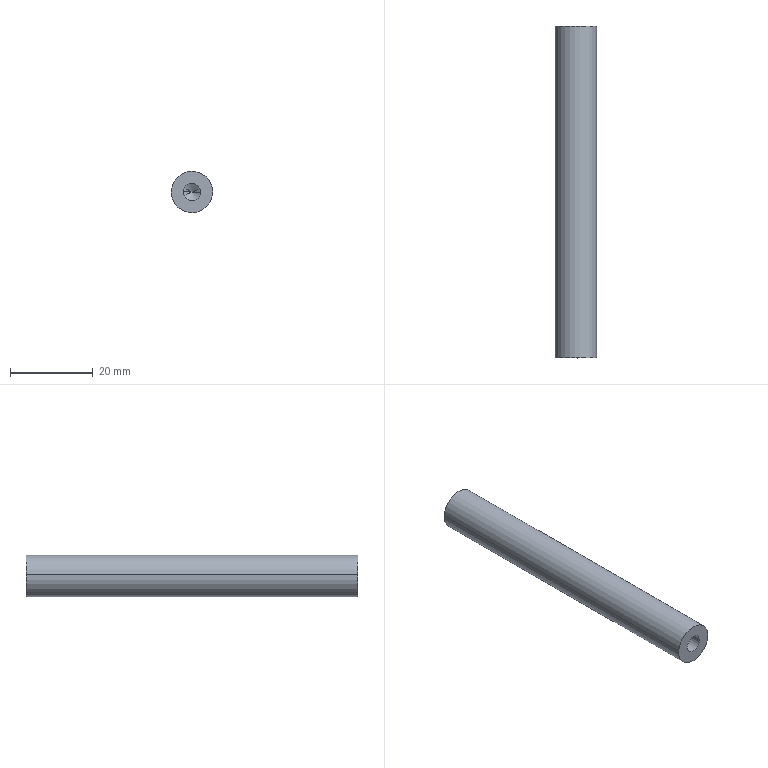Component | SolidWorks | 75-02-22MotorConnectingRod-1 | 1 solid | 12 faces | box 10 x 80 x 10 mm | volume 5928 mm3 | cylinder 6 | cone 4 | plane 2 | commonest cylinder face diameters 4.2 x4 10 x2 | material A3 Steel
build123d program:
from build123d import *

# Parameters (mm, degrees)
SKETCH1_R                       = 5
BOSS_EXTRUDE1_DEPTH             = 40
M5_TAPPED_HOLE1_D               = 4.2
M5_TAPPED_HOLE1_DEPTH           = 12.4
M5_TAPPED_HOLE1_TIP             = 1.262
M5_TAPPED_HOLE1_ON_FACE_2_D     = 4.2
M5_TAPPED_HOLE1_ON_FACE_2_DEPTH = 12.4
M5_TAPPED_HOLE1_ON_FACE_2_TIP   = 1.262


with BuildPart() as part:
    # Sketch1 → Boss-Extrude1 (new, symmetric)
    with BuildSketch(Plane.XY):
        Circle(SKETCH1_R)
    extrude(amount=BOSS_EXTRUDE1_DEPTH, both=True)

    # M5 Tapped Hole1
    with Locations(Plane.XY.offset(40)):
        with Locations((0, 0)):
            Hole(M5_TAPPED_HOLE1_D / 2, depth=M5_TAPPED_HOLE1_DEPTH)
            with Locations((0, 0, -(M5_TAPPED_HOLE1_DEPTH + M5_TAPPED_HOLE1_TIP / 2))):  # 118° drill point
                Cone(0, M5_TAPPED_HOLE1_D / 2, M5_TAPPED_HOLE1_TIP, mode=Mode.SUBTRACT)

    # M5 Tapped Hole1 on face 2
    with Locations(Plane(origin=(0, 0, -40), x_dir=(-1, 0, 0), z_dir=(0, 0, -1))):
        with Locations((0, 0)):
            Hole(M5_TAPPED_HOLE1_ON_FACE_2_D / 2, depth=M5_TAPPED_HOLE1_ON_FACE_2_DEPTH)
            with Locations((0, 0, -(M5_TAPPED_HOLE1_ON_FACE_2_DEPTH + M5_TAPPED_HOLE1_ON_FACE_2_TIP / 2))):  # 118° drill point
                Cone(0, M5_TAPPED_HOLE1_ON_FACE_2_D / 2, M5_TAPPED_HOLE1_ON_FACE_2_TIP, mode=Mode.SUBTRACT)


solid = part.part

# Placed as in the assembly
solid = solid.moved(Location((-17.8, 155.857, -17.75), (90, 0, 0)))
STEP:
#1=CARTESIAN_POINT('',(-0.6183,5.049,-0.7045));
#2=VERTEX_POINT('',#1);
#3=CARTESIAN_POINT('',(-0.7833,5.049,-0.6931));
#4=VERTEX_POINT('',#3);
#5=CARTESIAN_POINT('',(-0.7008,5.049,-0.6988));
#6=DIRECTION('',(-0.,-1.,0.));
#7=DIRECTION('',(-0.9976,0.,0.06881));
#8=AXIS2_PLACEMENT_3D('',#5,#6,#7);
#9=CIRCLE('',#8,0.08268);
#10=EDGE_CURVE('',#2,#4,#9,.T.);
#11=ORIENTED_EDGE('',*,*,#10,.F.);
#12=CARTESIAN_POINT('',(-0.6183,4.561,-0.7045));
#13=VERTEX_POINT('',#12);
#14=CARTESIAN_POINT('',(-0.6183,4.561,-0.7045));
#15=DIRECTION('',(-0.,-1.,0.));
#16=VECTOR('',#15,39.37);
#17=LINE('',#14,#16);
#18=EDGE_CURVE('',#2,#13,#17,.T.);
#19=ORIENTED_EDGE('',*,*,#18,.T.);
#20=CARTESIAN_POINT('',(-0.7833,4.561,-0.6931));
#21=VERTEX_POINT('',#20);
#22=CARTESIAN_POINT('',(-0.7008,4.561,-0.6988));
#23=DIRECTION('',(-0.,-1.,0.));
#24=DIRECTION('',(-0.9976,0.,0.06881));
#25=AXIS2_PLACEMENT_3D('',#22,#23,#24);
#26=CIRCLE('',#25,0.08268);
#27=EDGE_CURVE('',#13,#21,#26,.T.);
#28=ORIENTED_EDGE('',*,*,#27,.T.);
#29=CARTESIAN_POINT('',(-0.7833,4.561,-0.6931));
#30=DIRECTION('',(-0.,-1.,0.));
#31=VECTOR('',#30,39.37);
#32=LINE('',#29,#31);
#33=EDGE_CURVE('',#4,#21,#32,.T.);
#34=ORIENTED_EDGE('',*,*,#33,.F.);
#35=EDGE_LOOP('',(#11,#19,#28,#34));
#36=FACE_OUTER_BOUND('',#35,.T.);
#37=CARTESIAN_POINT('',(-0.7008,4.561,-0.6988));
#38=DIRECTION('',(-0.,-1.,0.));
#39=DIRECTION('',(-0.9976,0.,0.06881));
#40=AXIS2_PLACEMENT_3D('',#37,#38,#39);
#41=CYLINDRICAL_SURFACE('',#40,0.08268);
#42=ADVANCED_FACE('',(#36),#41,.F.);
#43=CARTESIAN_POINT('',(-0.7008,5.099,-0.6988));
#44=VERTEX_POINT('',#43);
#45=CARTESIAN_POINT('',(-0.7833,5.049,-0.6931));
#46=DIRECTION('',(-0.8551,-0.515,0.05899));
#47=VECTOR('',#46,39.37);
#48=LINE('',#45,#47);
#49=EDGE_CURVE('',#44,#4,#48,.T.);
#50=ORIENTED_EDGE('',*,*,#49,.F.);
#51=CARTESIAN_POINT('',(-0.6183,5.049,-0.7045));
#52=DIRECTION('',(0.8551,-0.515,-0.05899));
#53=VECTOR('',#52,39.37);
#54=LINE('',#51,#53);
#55=EDGE_CURVE('',#44,#2,#54,.T.);
#56=ORIENTED_EDGE('',*,*,#55,.T.);
#57=ORIENTED_EDGE('',*,*,#10,.T.);
#58=EDGE_LOOP('',(#50,#56,#57));
#59=FACE_OUTER_BOUND('',#58,.T.);
#60=CARTESIAN_POINT('',(-0.7008,5.049,-0.6988));
#61=DIRECTION('',(-0.,-1.,0.));
#62=DIRECTION('',(-0.9976,0.,0.06881));
#63=AXIS2_PLACEMENT_3D('',#60,#61,#62);
#64=CONICAL_SURFACE('',#63,0.08268,1.03);
#65=ADVANCED_FACE('',(#59),#64,.F.);
#66=CARTESIAN_POINT('',(-0.7833,7.223,-0.6931));
#67=VERTEX_POINT('',#66);
#68=CARTESIAN_POINT('',(-0.6183,7.223,-0.7045));
#69=VERTEX_POINT('',#68);
#70=CARTESIAN_POINT('',(-0.7008,7.223,-0.6988));
#71=DIRECTION('',(0.,1.,-0.));
#72=DIRECTION('',(0.9976,0.,-0.06881));
#73=AXIS2_PLACEMENT_3D('',#70,#71,#72);
#74=CIRCLE('',#73,0.08268);
#75=EDGE_CURVE('',#67,#69,#74,.T.);
#76=ORIENTED_EDGE('',*,*,#75,.F.);
#77=CARTESIAN_POINT('',(-0.7833,7.711,-0.6931));
#78=VERTEX_POINT('',#77);
#79=CARTESIAN_POINT('',(-0.7833,7.711,-0.6931));
#80=DIRECTION('',(0.,1.,-0.));
#81=VECTOR('',#80,39.37);
#82=LINE('',#79,#81);
#83=EDGE_CURVE('',#67,#78,#82,.T.);
#84=ORIENTED_EDGE('',*,*,#83,.T.);
#85=CARTESIAN_POINT('',(-0.6183,7.711,-0.7045));
#86=VERTEX_POINT('',#85);
#87=CARTESIAN_POINT('',(-0.7008,7.711,-0.6988));
#88=DIRECTION('',(0.,1.,-0.));
#89=DIRECTION('',(0.9976,0.,-0.06881));
#90=AXIS2_PLACEMENT_3D('',#87,#88,#89);
#91=CIRCLE('',#90,0.08268);
#92=EDGE_CURVE('',#78,#86,#91,.T.);
#93=ORIENTED_EDGE('',*,*,#92,.T.);
#94=CARTESIAN_POINT('',(-0.6183,7.711,-0.7045));
#95=DIRECTION('',(0.,1.,-0.));
#96=VECTOR('',#95,39.37);
#97=LINE('',#94,#96);
#98=EDGE_CURVE('',#69,#86,#97,.T.);
#99=ORIENTED_EDGE('',*,*,#98,.F.);
#100=EDGE_LOOP('',(#76,#84,#93,#99));
#101=FACE_OUTER_BOUND('',#100,.T.);
#102=CARTESIAN_POINT('',(-0.7008,7.711,-0.6988));
#103=DIRECTION('',(0.,1.,-0.));
#104=DIRECTION('',(0.9976,0.,-0.06881));
#105=AXIS2_PLACEMENT_3D('',#102,#103,#104);
#106=CYLINDRICAL_SURFACE('',#105,0.08268);
#107=ADVANCED_FACE('',(#101),#106,.F.);
#108=CARTESIAN_POINT('',(-0.7008,7.173,-0.6988));
#109=VERTEX_POINT('',#108);
#110=CARTESIAN_POINT('',(-0.6183,7.223,-0.7045));
#111=DIRECTION('',(0.8551,0.515,-0.05899));
#112=VECTOR('',#111,39.37);
#113=LINE('',#110,#112);
#114=EDGE_CURVE('',#109,#69,#113,.T.);
#115=ORIENTED_EDGE('',*,*,#114,.F.);
#116=CARTESIAN_POINT('',(-0.7833,7.223,-0.6931));
#117=DIRECTION('',(-0.8551,0.515,0.05899));
#118=VECTOR('',#117,39.37);
#119=LINE('',#116,#118);
#120=EDGE_CURVE('',#109,#67,#119,.T.);
#121=ORIENTED_EDGE('',*,*,#120,.T.);
#122=ORIENTED_EDGE('',*,*,#75,.T.);
#123=EDGE_LOOP('',(#115,#121,#122));
#124=FACE_OUTER_BOUND('',#123,.T.);
#125=CARTESIAN_POINT('',(-0.7008,7.223,-0.6988));
#126=DIRECTION('',(0.,1.,-0.));
#127=DIRECTION('',(0.9976,0.,-0.06881));
#128=AXIS2_PLACEMENT_3D('',#125,#126,#127);
#129=CONICAL_SURFACE('',#128,0.08268,1.03);
#130=ADVANCED_FACE('',(#124),#129,.F.);
#131=CARTESIAN_POINT('',(-0.8972,4.561,-0.6853));
#132=VERTEX_POINT('',#131);
#133=CARTESIAN_POINT('',(-0.5044,4.561,-0.7124));
#134=VERTEX_POINT('',#133);
#135=CARTESIAN_POINT('',(-0.7008,4.561,-0.6988));
#136=DIRECTION('',(-0.,-1.,0.));
#137=DIRECTION('',(-0.9976,0.,0.06881));
#138=AXIS2_PLACEMENT_3D('',#135,#136,#137);
#139=CIRCLE('',#138,0.1969);
#140=EDGE_CURVE('',#132,#134,#139,.T.);
#141=ORIENTED_EDGE('',*,*,#140,.F.);
#142=CARTESIAN_POINT('',(-0.8972,7.711,-0.6853));
#143=VERTEX_POINT('',#142);
#144=CARTESIAN_POINT('',(-0.8972,4.561,-0.6853));
#145=DIRECTION('',(0.,1.,-0.));
#146=VECTOR('',#145,39.37);
#147=LINE('',#144,#146);
#148=EDGE_CURVE('',#132,#143,#147,.T.);
#149=ORIENTED_EDGE('',*,*,#148,.T.);
#150=CARTESIAN_POINT('',(-0.5044,7.711,-0.7124));
#151=VERTEX_POINT('',#150);
#152=CARTESIAN_POINT('',(-0.7008,7.711,-0.6988));
#153=DIRECTION('',(-0.,-1.,0.));
#154=DIRECTION('',(-0.9976,0.,0.06881));
#155=AXIS2_PLACEMENT_3D('',#152,#153,#154);
#156=CIRCLE('',#155,0.1969);
#157=EDGE_CURVE('',#143,#151,#156,.T.);
#158=ORIENTED_EDGE('',*,*,#157,.T.);
#159=CARTESIAN_POINT('',(-0.5044,4.561,-0.7124));
#160=DIRECTION('',(0.,1.,-0.));
#161=VECTOR('',#160,39.37);
#162=LINE('',#159,#161);
#163=EDGE_CURVE('',#134,#151,#162,.T.);
#164=ORIENTED_EDGE('',*,*,#163,.F.);
#165=EDGE_LOOP('',(#141,#149,#158,#164));
#166=FACE_OUTER_BOUND('',#165,.T.);
#167=CARTESIAN_POINT('',(-0.7008,4.561,-0.6988));
#168=DIRECTION('',(0.,1.,-0.));
#169=DIRECTION('',(0.9976,0.,-0.06881));
#170=AXIS2_PLACEMENT_3D('',#167,#168,#169);
#171=CYLINDRICAL_SURFACE('',#170,0.1969);
#172=ADVANCED_FACE('',(#166),#171,.T.);
#173=ORIENTED_EDGE('',*,*,#148,.F.);
#174=CARTESIAN_POINT('',(-0.7008,4.561,-0.6988));
#175=DIRECTION('',(-0.,-1.,0.));
#176=DIRECTION('',(-0.9976,0.,0.06881));
#177=AXIS2_PLACEMENT_3D('',#174,#175,#176);
#178=CIRCLE('',#177,0.1969);
#179=EDGE_CURVE('',#134,#132,#178,.T.);
#180=ORIENTED_EDGE('',*,*,#179,.F.);
#181=ORIENTED_EDGE('',*,*,#163,.T.);
#182=CARTESIAN_POINT('',(-0.7008,7.711,-0.6988));
#183=DIRECTION('',(-0.,-1.,0.));
#184=DIRECTION('',(-0.9976,0.,0.06881));
#185=AXIS2_PLACEMENT_3D('',#182,#183,#184);
#186=CIRCLE('',#185,0.1969);
#187=EDGE_CURVE('',#151,#143,#186,.T.);
#188=ORIENTED_EDGE('',*,*,#187,.T.);
#189=EDGE_LOOP('',(#173,#180,#181,#188));
#190=FACE_OUTER_BOUND('',#189,.T.);
#191=CARTESIAN_POINT('',(-0.7008,4.561,-0.6988));
#192=DIRECTION('',(0.,1.,-0.));
#193=DIRECTION('',(0.9976,0.,-0.06881));
#194=AXIS2_PLACEMENT_3D('',#191,#192,#193);
#195=CYLINDRICAL_SURFACE('',#194,0.1969);
#196=ADVANCED_FACE('',(#190),#195,.T.);
#197=CARTESIAN_POINT('',(-0.7008,4.561,-0.6988));
#198=DIRECTION('',(-0.,-1.,0.));
#199=DIRECTION('',(-0.9976,0.,0.06881));
#200=AXIS2_PLACEMENT_3D('',#197,#198,#199);
#201=CIRCLE('',#200,0.08268);
#202=EDGE_CURVE('',#21,#13,#201,.T.);
#203=ORIENTED_EDGE('',*,*,#202,.F.);
#204=ORIENTED_EDGE('',*,*,#27,.F.);
#205=EDGE_LOOP('',(#203,#204));
#206=FACE_BOUND('',#205,.T.);
#207=ORIENTED_EDGE('',*,*,#179,.T.);
#208=ORIENTED_EDGE('',*,*,#140,.T.);
#209=EDGE_LOOP('',(#207,#208));
#210=FACE_OUTER_BOUND('',#209,.T.);
#211=CARTESIAN_POINT('',(-0.7008,4.561,-0.6988));
#212=DIRECTION('',(-0.,-1.,0.));
#213=DIRECTION('',(-0.9976,0.,0.06881));
#214=AXIS2_PLACEMENT_3D('',#211,#212,#213);
#215=PLANE('',#214);
#216=ADVANCED_FACE('',(#206,#210),#215,.T.);
#217=CARTESIAN_POINT('',(-0.7008,7.711,-0.6988));
#218=DIRECTION('',(0.,1.,-0.));
#219=DIRECTION('',(0.9976,0.,-0.06881));
#220=AXIS2_PLACEMENT_3D('',#217,#218,#219);
#221=CIRCLE('',#220,0.08268);
#222=EDGE_CURVE('',#86,#78,#221,.T.);
#223=ORIENTED_EDGE('',*,*,#222,.F.);
#224=ORIENTED_EDGE('',*,*,#92,.F.);
#225=EDGE_LOOP('',(#223,#224));
#226=FACE_BOUND('',#225,.T.);
#227=ORIENTED_EDGE('',*,*,#187,.F.);
#228=ORIENTED_EDGE('',*,*,#157,.F.);
#229=EDGE_LOOP('',(#227,#228));
#230=FACE_OUTER_BOUND('',#229,.T.);
#231=CARTESIAN_POINT('',(-0.7008,7.711,-0.6988));
#232=DIRECTION('',(-0.,-1.,0.));
#233=DIRECTION('',(-0.9976,0.,0.06881));
#234=AXIS2_PLACEMENT_3D('',#231,#232,#233);
#235=PLANE('',#234);
#236=ADVANCED_FACE('',(#226,#230),#235,.F.);
#237=ORIENTED_EDGE('',*,*,#120,.F.);
#238=ORIENTED_EDGE('',*,*,#114,.T.);
#239=CARTESIAN_POINT('',(-0.7008,7.223,-0.6988));
#240=DIRECTION('',(0.,1.,-0.));
#241=DIRECTION('',(0.9976,0.,-0.06881));
#242=AXIS2_PLACEMENT_3D('',#239,#240,#241);
#243=CIRCLE('',#242,0.08268);
#244=EDGE_CURVE('',#69,#67,#243,.T.);
#245=ORIENTED_EDGE('',*,*,#244,.T.);
#246=EDGE_LOOP('',(#237,#238,#245));
#247=FACE_OUTER_BOUND('',#246,.T.);
#248=CARTESIAN_POINT('',(-0.7008,7.223,-0.6988));
#249=DIRECTION('',(0.,1.,-0.));
#250=DIRECTION('',(0.9976,0.,-0.06881));
#251=AXIS2_PLACEMENT_3D('',#248,#249,#250);
#252=CONICAL_SURFACE('',#251,0.08268,1.03);
#253=ADVANCED_FACE('',(#247),#252,.F.);
#254=ORIENTED_EDGE('',*,*,#83,.F.);
#255=ORIENTED_EDGE('',*,*,#244,.F.);
#256=ORIENTED_EDGE('',*,*,#98,.T.);
#257=ORIENTED_EDGE('',*,*,#222,.T.);
#258=EDGE_LOOP('',(#254,#255,#256,#257));
#259=FACE_OUTER_BOUND('',#258,.T.);
#260=CARTESIAN_POINT('',(-0.7008,7.711,-0.6988));
#261=DIRECTION('',(0.,1.,-0.));
#262=DIRECTION('',(0.9976,0.,-0.06881));
#263=AXIS2_PLACEMENT_3D('',#260,#261,#262);
#264=CYLINDRICAL_SURFACE('',#263,0.08268);
#265=ADVANCED_FACE('',(#259),#264,.F.);
#266=ORIENTED_EDGE('',*,*,#55,.F.);
#267=ORIENTED_EDGE('',*,*,#49,.T.);
#268=CARTESIAN_POINT('',(-0.7008,5.049,-0.6988));
#269=DIRECTION('',(-0.,-1.,0.));
#270=DIRECTION('',(-0.9976,0.,0.06881));
#271=AXIS2_PLACEMENT_3D('',#268,#269,#270);
#272=CIRCLE('',#271,0.08268);
#273=EDGE_CURVE('',#4,#2,#272,.T.);
#274=ORIENTED_EDGE('',*,*,#273,.T.);
#275=EDGE_LOOP('',(#266,#267,#274));
#276=FACE_OUTER_BOUND('',#275,.T.);
#277=CARTESIAN_POINT('',(-0.7008,5.049,-0.6988));
#278=DIRECTION('',(-0.,-1.,0.));
#279=DIRECTION('',(-0.9976,0.,0.06881));
#280=AXIS2_PLACEMENT_3D('',#277,#278,#279);
#281=CONICAL_SURFACE('',#280,0.08268,1.03);
#282=ADVANCED_FACE('',(#276),#281,.F.);
#283=ORIENTED_EDGE('',*,*,#18,.F.);
#284=ORIENTED_EDGE('',*,*,#273,.F.);
#285=ORIENTED_EDGE('',*,*,#33,.T.);
#286=ORIENTED_EDGE('',*,*,#202,.T.);
#287=EDGE_LOOP('',(#283,#284,#285,#286));
#288=FACE_OUTER_BOUND('',#287,.T.);
#289=CARTESIAN_POINT('',(-0.7008,4.561,-0.6988));
#290=DIRECTION('',(-0.,-1.,0.));
#291=DIRECTION('',(-0.9976,0.,0.06881));
#292=AXIS2_PLACEMENT_3D('',#289,#290,#291);
#293=CYLINDRICAL_SURFACE('',#292,0.08268);
#294=ADVANCED_FACE('',(#288),#293,.F.);
#295=CLOSED_SHELL('',(#42,#65,#107,#130,#172,#196,#216,#236,#253,#265,#282,#294));
#296=MANIFOLD_SOLID_BREP('',#295);
#297=CARTESIAN_POINT('',(0.,0.,0.));
#298=DIRECTION('',(0.,0.,1.));
#299=DIRECTION('',(1.,0.,0.));
#300=AXIS2_PLACEMENT_3D('',#297,#298,#299);
#301=(LENGTH_UNIT()NAMED_UNIT(*)SI_UNIT($,.METRE.));
#302=LENGTH_MEASURE_WITH_UNIT(LENGTH_MEASURE(0.0254),#301);
#303=DIMENSIONAL_EXPONENTS(1.,0.,0.,0.,0.,0.,0.);
#304=(CONVERSION_BASED_UNIT('',#302)LENGTH_UNIT()NAMED_UNIT(#303));
#305=UNCERTAINTY_MEASURE_WITH_UNIT(LENGTH_MEASURE(0.00001),#304,'','');
#306=(NAMED_UNIT(*)PLANE_ANGLE_UNIT()SI_UNIT($,.RADIAN.));
#307=(NAMED_UNIT(*)SI_UNIT($,.STERADIAN.)SOLID_ANGLE_UNIT());
#308=(GEOMETRIC_REPRESENTATION_CONTEXT(3)GLOBAL_UNCERTAINTY_ASSIGNED_CONTEXT((#305))GLOBAL_UNIT_ASSIGNED_CONTEXT((#304,#306,#307))REPRESENTATION_CONTEXT('',''));
#309=ADVANCED_BREP_SHAPE_REPRESENTATION('',(#296,#300),#308);
#310=COLOUR_RGB('',0.7922,0.8196,0.9333);
#311=FILL_AREA_STYLE_COLOUR('',#310);
#312=FILL_AREA_STYLE('',(#311));
#313=SURFACE_STYLE_FILL_AREA(#312);
#314=SURFACE_SIDE_STYLE('',(#313));
#315=SURFACE_STYLE_USAGE(.BOTH.,#314);
#316=PRESENTATION_STYLE_ASSIGNMENT((#315));
#317=STYLED_ITEM('',(#316),#296);
#318=PRESENTATION_LAYER_ASSIGNMENT('','',(#317));
#319=(LENGTH_UNIT()NAMED_UNIT(*)SI_UNIT($,.METRE.));
#320=LENGTH_MEASURE_WITH_UNIT(LENGTH_MEASURE(0.0254),#319);
#321=DIMENSIONAL_EXPONENTS(1.,0.,0.,0.,0.,0.,0.);
#322=(CONVERSION_BASED_UNIT('',#320)LENGTH_UNIT()NAMED_UNIT(#321));
#323=UNCERTAINTY_MEASURE_WITH_UNIT(LENGTH_MEASURE(0.00001),#322,'','');
#324=(NAMED_UNIT(*)PLANE_ANGLE_UNIT()SI_UNIT($,.RADIAN.));
#325=(NAMED_UNIT(*)SI_UNIT($,.STERADIAN.)SOLID_ANGLE_UNIT());
#326=(GEOMETRIC_REPRESENTATION_CONTEXT(3)GLOBAL_UNCERTAINTY_ASSIGNED_CONTEXT((#323))GLOBAL_UNIT_ASSIGNED_CONTEXT((#322,#324,#325))REPRESENTATION_CONTEXT('',''));
#327=MECHANICAL_DESIGN_GEOMETRIC_PRESENTATION_REPRESENTATION('',(#317),#326);